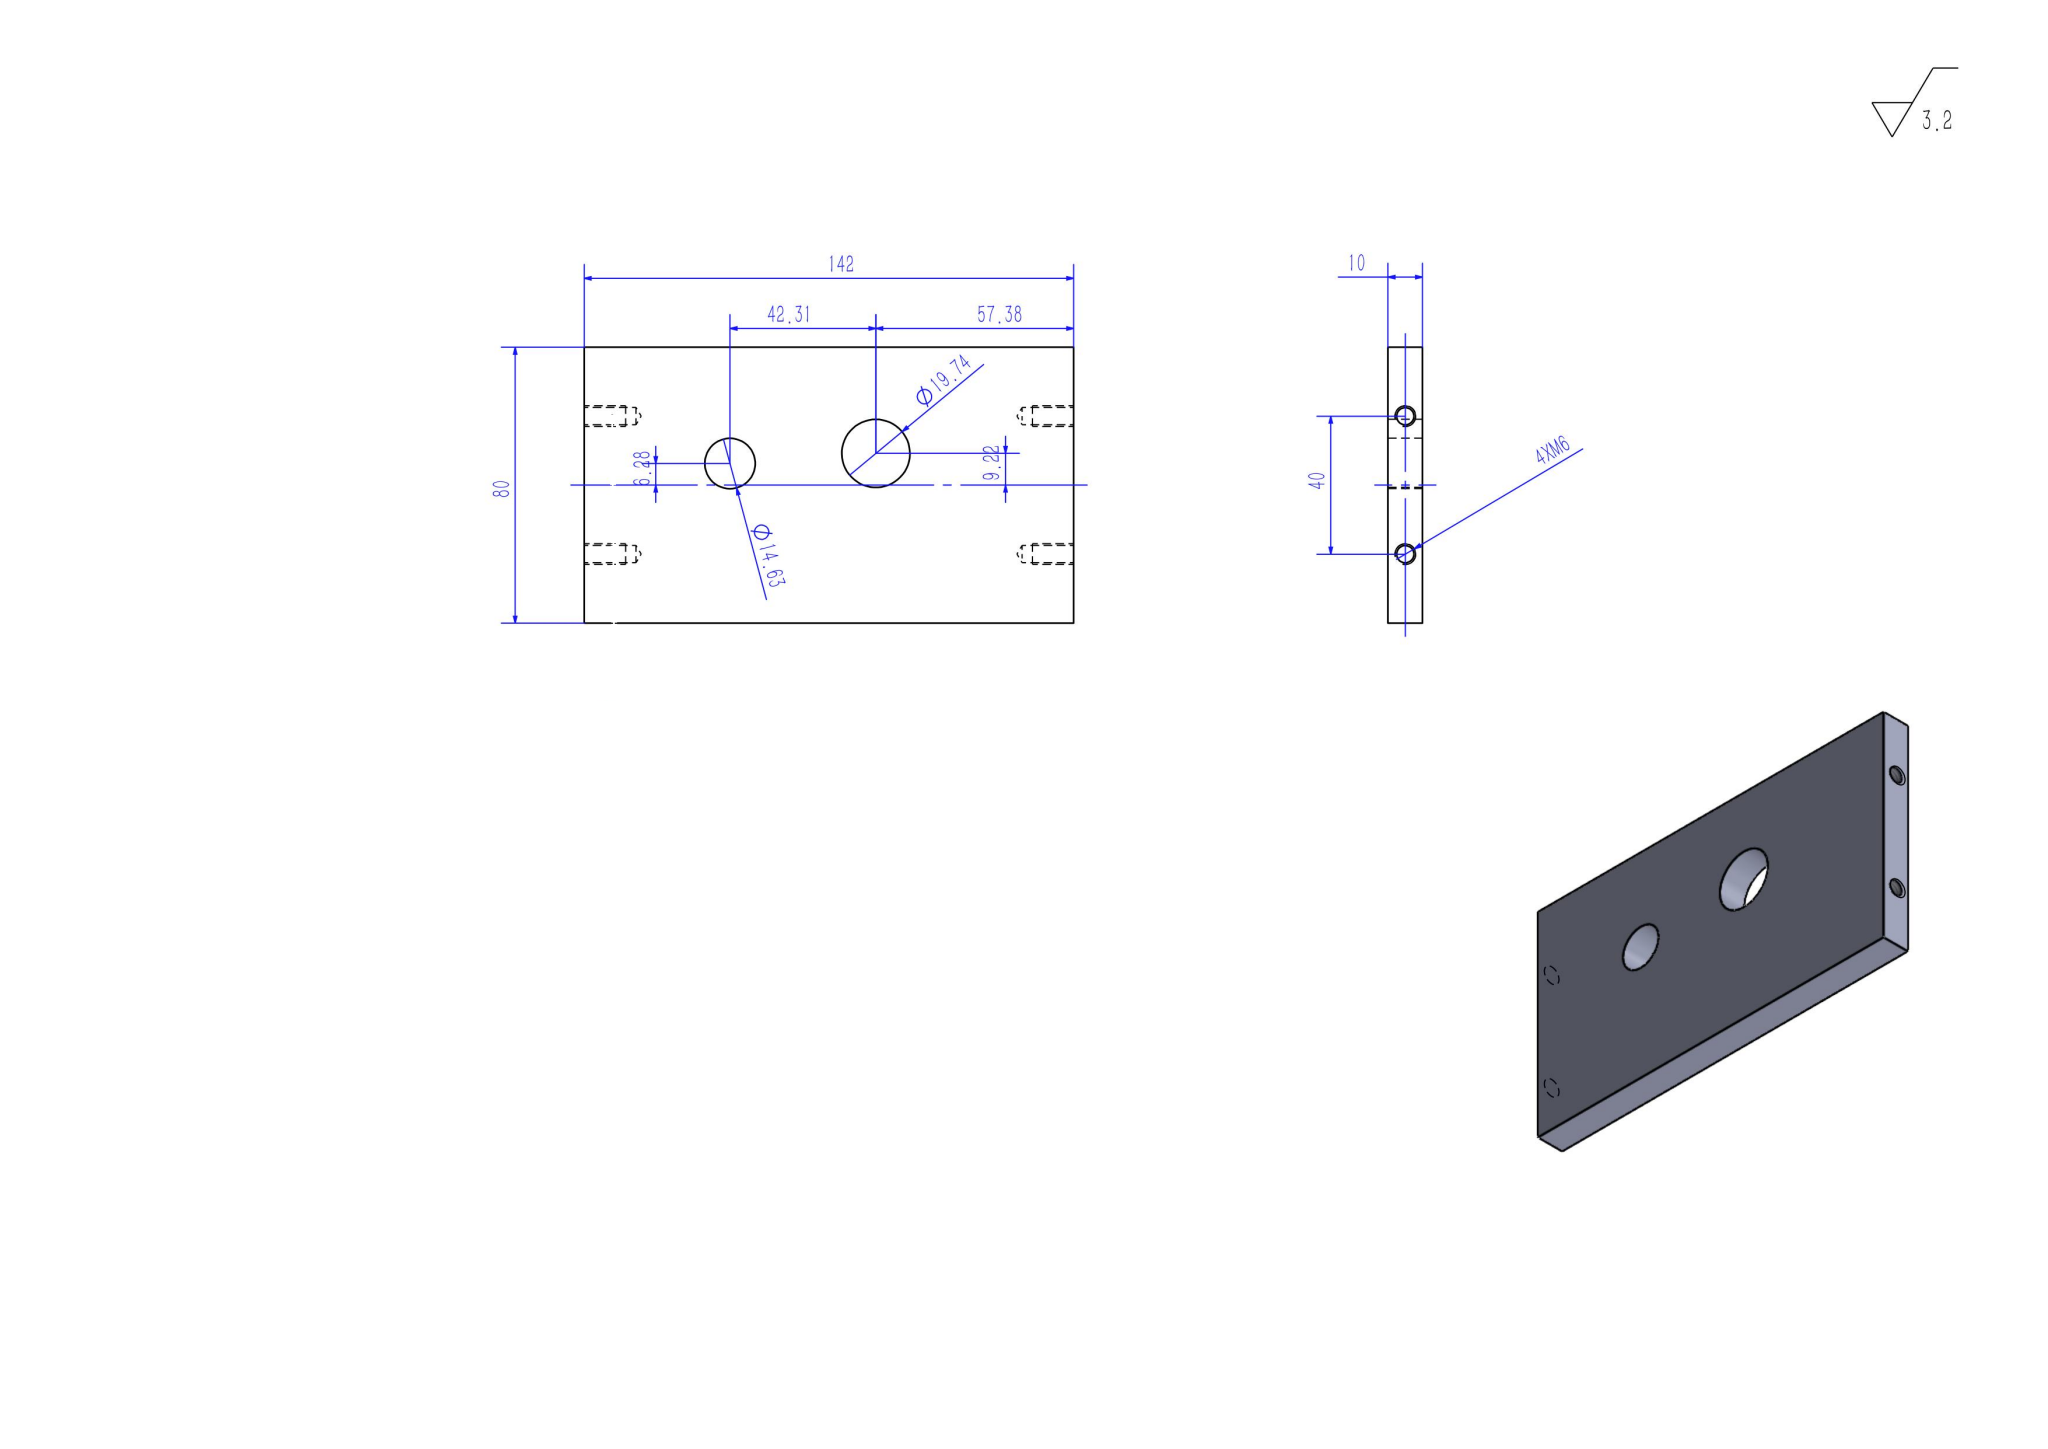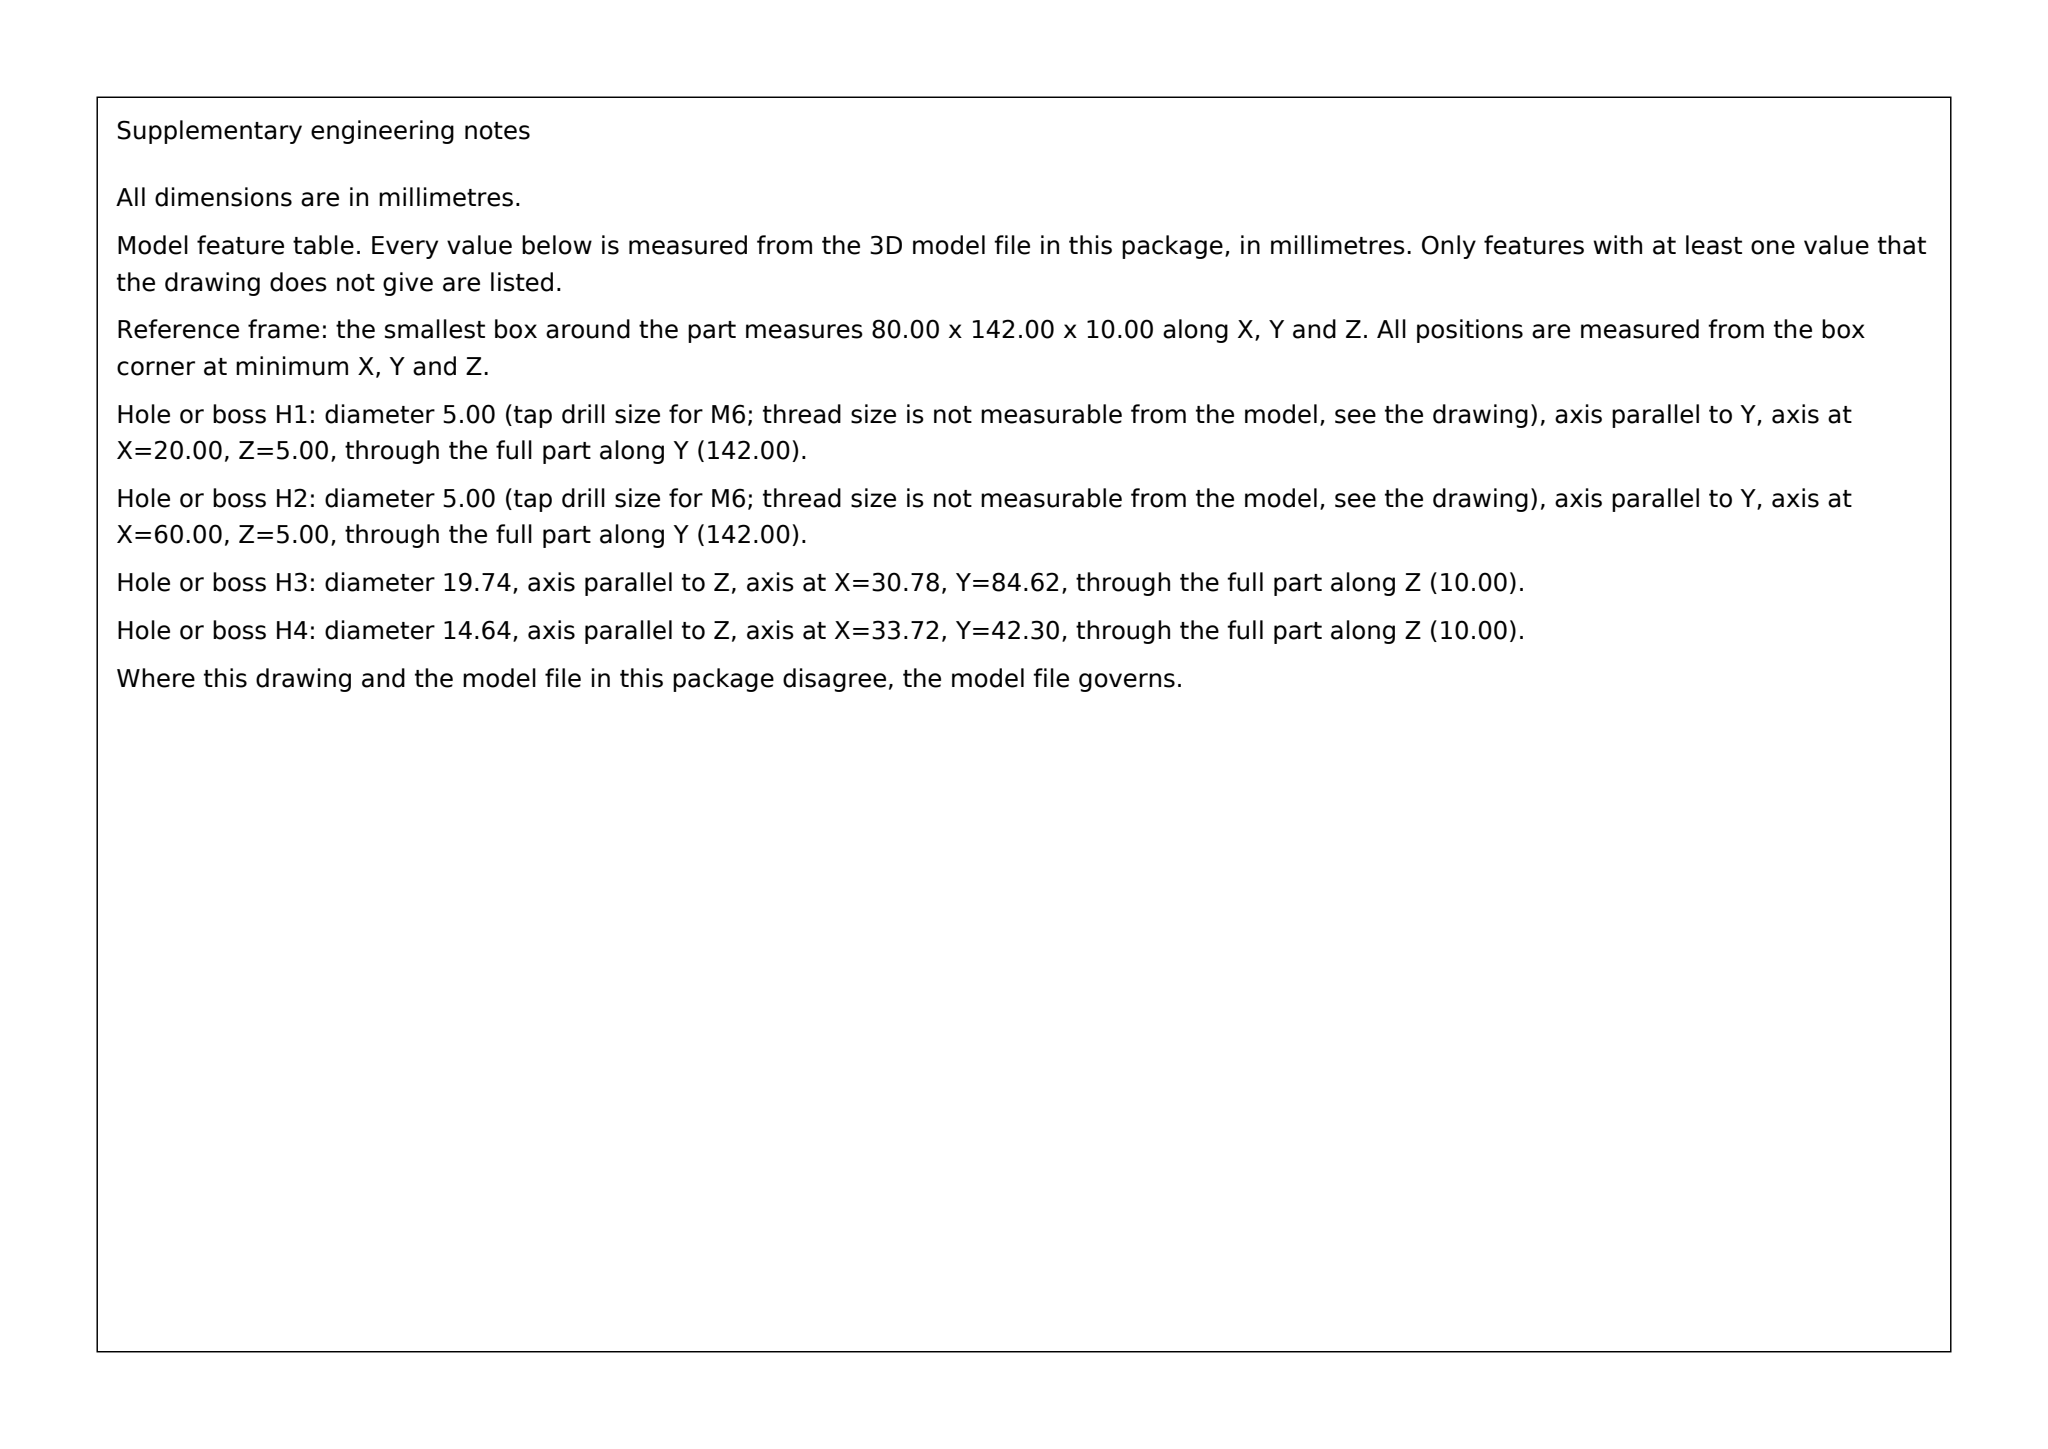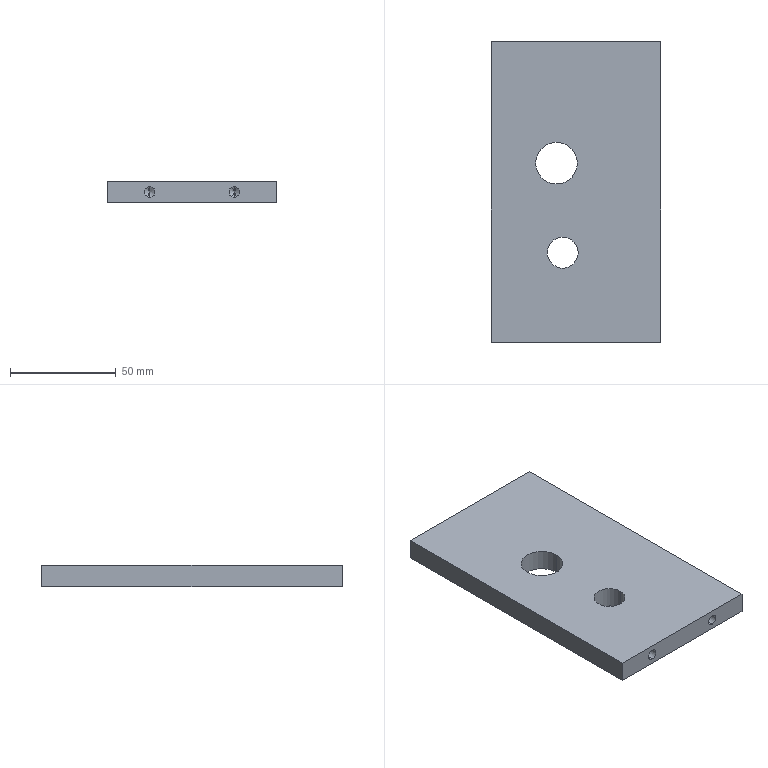Part | SolidWorks | mm | 1 solid | 26 faces | box 80 x 142 x 10 mm | volume 107639 mm3 | cylinder 12 | cone 8 | plane 6 | commonest cylinder face diameters 5 x8 14.633 x2 19.744 x2
build123d program:
from build123d import *

# Parameters (mm, degrees)
SKETCH1_W             = 80
SKETCH1_H             = 10
BOSS_EXTRUDE1_DEPTH   = 71
M6_TAPPED_HOLE1_D     = 5
M6_TAPPED_HOLE1_DEPTH = 15
M6_TAPPED_HOLE1_TIP   = 1.502
M6_TAPPED_HOLE2_D     = 5
M6_TAPPED_HOLE2_DEPTH = 15
M6_TAPPED_HOLE2_TIP   = 1.502
SKETCH6_R             = 7.317
SKETCH6_R_2           = 9.872
CUT_EXTRUDE1_DEPTH    = 80


with BuildPart() as part:
    # Sketch1 → Boss-Extrude1 (new, symmetric)
    with BuildSketch(Plane(origin=(0, 0, 0), x_dir=(1, 0, 0), z_dir=(0, 1, 0))):
        Rectangle(SKETCH1_W, SKETCH1_H)
    extrude(amount=BOSS_EXTRUDE1_DEPTH, both=True)

    # M6 Tapped Hole1
    with Locations(Plane(origin=(0, -71, 0), x_dir=(-1, 0, 0), z_dir=(0, -1, 0))):
        with Locations((20, 0), (-20, 0)):
            Hole(M6_TAPPED_HOLE1_D / 2, depth=M6_TAPPED_HOLE1_DEPTH)
            with Locations((0, 0, -(M6_TAPPED_HOLE1_DEPTH + M6_TAPPED_HOLE1_TIP / 2))):  # 118° drill point
                Cone(0, M6_TAPPED_HOLE1_D / 2, M6_TAPPED_HOLE1_TIP, mode=Mode.SUBTRACT)

    # M6 Tapped Hole2
    with Locations(Plane(origin=(0, 71, 0), x_dir=(1, 0, 0), z_dir=(0, 1, 0))):
        with Locations((-20, 0), (20, 0)):
            Hole(M6_TAPPED_HOLE2_D / 2, depth=M6_TAPPED_HOLE2_DEPTH)
            with Locations((0, 0, -(M6_TAPPED_HOLE2_DEPTH + M6_TAPPED_HOLE2_TIP / 2))):  # 118° drill point
                Cone(0, M6_TAPPED_HOLE2_D / 2, M6_TAPPED_HOLE2_TIP, mode=Mode.SUBTRACT)

    # Sketch6 → Cut-Extrude1 (cut)
    with BuildSketch(Plane(origin=(0, 0, -5), x_dir=(-1, 0, 0), z_dir=(0, 0, -1))):
        with Locations((6.284, -28.698)):
            Circle(SKETCH6_R)
        with Locations((9.217, 13.616)):
            Circle(SKETCH6_R_2)
    extrude(amount=-CUT_EXTRUDE1_DEPTH, mode=Mode.SUBTRACT)


solid = part.part
STEP:
#1=CARTESIAN_POINT('',(1.032,-28.698,5.));
#2=VERTEX_POINT('',#1);
#3=CARTESIAN_POINT('',(-13.601,-28.698,5.));
#4=VERTEX_POINT('',#3);
#5=CARTESIAN_POINT('',(-6.284,-28.698,5.));
#6=DIRECTION('',(0.,0.,-1.));
#7=DIRECTION('',(-1.,0.,0.));
#8=AXIS2_PLACEMENT_3D('',#5,#6,#7);
#9=CIRCLE('',#8,7.317);
#10=EDGE_CURVE('',#2,#4,#9,.T.);
#11=ORIENTED_EDGE('',*,*,#10,.F.);
#12=CARTESIAN_POINT('',(1.032,-28.698,-5.));
#13=VERTEX_POINT('',#12);
#14=CARTESIAN_POINT('',(1.032,-28.698,75.));
#15=DIRECTION('',(0.,0.,-1.));
#16=VECTOR('',#15,1000.);
#17=LINE('',#14,#16);
#18=EDGE_CURVE('',#2,#13,#17,.T.);
#19=ORIENTED_EDGE('',*,*,#18,.T.);
#20=CARTESIAN_POINT('',(-13.601,-28.698,-5.));
#21=VERTEX_POINT('',#20);
#22=CARTESIAN_POINT('',(-6.284,-28.698,-5.));
#23=DIRECTION('',(0.,0.,-1.));
#24=DIRECTION('',(-1.,0.,0.));
#25=AXIS2_PLACEMENT_3D('',#22,#23,#24);
#26=CIRCLE('',#25,7.317);
#27=EDGE_CURVE('',#13,#21,#26,.T.);
#28=ORIENTED_EDGE('',*,*,#27,.T.);
#29=CARTESIAN_POINT('',(-13.601,-28.698,75.));
#30=DIRECTION('',(0.,0.,-1.));
#31=VECTOR('',#30,1000.);
#32=LINE('',#29,#31);
#33=EDGE_CURVE('',#4,#21,#32,.T.);
#34=ORIENTED_EDGE('',*,*,#33,.F.);
#35=EDGE_LOOP('',(#11,#19,#28,#34));
#36=FACE_OUTER_BOUND('',#35,.T.);
#37=CARTESIAN_POINT('',(-6.284,-28.698,75.));
#38=DIRECTION('',(0.,0.,-1.));
#39=DIRECTION('',(-1.,0.,0.));
#40=AXIS2_PLACEMENT_3D('',#37,#38,#39);
#41=CYLINDRICAL_SURFACE('',#40,7.317);
#42=ADVANCED_FACE('',(#36),#41,.F.);
#43=CARTESIAN_POINT('',(0.6551,13.616,5.));
#44=VERTEX_POINT('',#43);
#45=CARTESIAN_POINT('',(-19.089,13.616,5.));
#46=VERTEX_POINT('',#45);
#47=CARTESIAN_POINT('',(-9.217,13.616,5.));
#48=DIRECTION('',(0.,0.,-1.));
#49=DIRECTION('',(-1.,0.,0.));
#50=AXIS2_PLACEMENT_3D('',#47,#48,#49);
#51=CIRCLE('',#50,9.872);
#52=EDGE_CURVE('',#44,#46,#51,.T.);
#53=ORIENTED_EDGE('',*,*,#52,.F.);
#54=CARTESIAN_POINT('',(0.6551,13.616,-5.));
#55=VERTEX_POINT('',#54);
#56=CARTESIAN_POINT('',(0.6551,13.616,75.));
#57=DIRECTION('',(0.,0.,-1.));
#58=VECTOR('',#57,1000.);
#59=LINE('',#56,#58);
#60=EDGE_CURVE('',#44,#55,#59,.T.);
#61=ORIENTED_EDGE('',*,*,#60,.T.);
#62=CARTESIAN_POINT('',(-19.089,13.616,-5.));
#63=VERTEX_POINT('',#62);
#64=CARTESIAN_POINT('',(-9.217,13.616,-5.));
#65=DIRECTION('',(0.,0.,-1.));
#66=DIRECTION('',(-1.,0.,0.));
#67=AXIS2_PLACEMENT_3D('',#64,#65,#66);
#68=CIRCLE('',#67,9.872);
#69=EDGE_CURVE('',#55,#63,#68,.T.);
#70=ORIENTED_EDGE('',*,*,#69,.T.);
#71=CARTESIAN_POINT('',(-19.089,13.616,75.));
#72=DIRECTION('',(0.,0.,-1.));
#73=VECTOR('',#72,1000.);
#74=LINE('',#71,#73);
#75=EDGE_CURVE('',#46,#63,#74,.T.);
#76=ORIENTED_EDGE('',*,*,#75,.F.);
#77=EDGE_LOOP('',(#53,#61,#70,#76));
#78=FACE_OUTER_BOUND('',#77,.T.);
#79=CARTESIAN_POINT('',(-9.217,13.616,75.));
#80=DIRECTION('',(0.,0.,-1.));
#81=DIRECTION('',(-1.,0.,0.));
#82=AXIS2_PLACEMENT_3D('',#79,#80,#81);
#83=CYLINDRICAL_SURFACE('',#82,9.872);
#84=ADVANCED_FACE('',(#78),#83,.F.);
#85=CARTESIAN_POINT('',(-20.,56.,-2.5));
#86=VERTEX_POINT('',#85);
#87=CARTESIAN_POINT('',(-20.,56.,2.5));
#88=VERTEX_POINT('',#87);
#89=CARTESIAN_POINT('',(-20.,56.,0.));
#90=DIRECTION('',(0.,1.,0.));
#91=DIRECTION('',(0.,0.,1.));
#92=AXIS2_PLACEMENT_3D('',#89,#90,#91);
#93=CIRCLE('',#92,2.5);
#94=EDGE_CURVE('',#86,#88,#93,.T.);
#95=ORIENTED_EDGE('',*,*,#94,.F.);
#96=CARTESIAN_POINT('',(-20.,71.,-2.5));
#97=VERTEX_POINT('',#96);
#98=CARTESIAN_POINT('',(-20.,71.,-2.5));
#99=DIRECTION('',(0.,1.,0.));
#100=VECTOR('',#99,1000.);
#101=LINE('',#98,#100);
#102=EDGE_CURVE('',#86,#97,#101,.T.);
#103=ORIENTED_EDGE('',*,*,#102,.T.);
#104=CARTESIAN_POINT('',(-20.,71.,2.5));
#105=VERTEX_POINT('',#104);
#106=CARTESIAN_POINT('',(-20.,71.,0.));
#107=DIRECTION('',(0.,1.,0.));
#108=DIRECTION('',(0.,0.,1.));
#109=AXIS2_PLACEMENT_3D('',#106,#107,#108);
#110=CIRCLE('',#109,2.5);
#111=EDGE_CURVE('',#97,#105,#110,.T.);
#112=ORIENTED_EDGE('',*,*,#111,.T.);
#113=CARTESIAN_POINT('',(-20.,71.,2.5));
#114=DIRECTION('',(0.,1.,0.));
#115=VECTOR('',#114,1000.);
#116=LINE('',#113,#115);
#117=EDGE_CURVE('',#88,#105,#116,.T.);
#118=ORIENTED_EDGE('',*,*,#117,.F.);
#119=EDGE_LOOP('',(#95,#103,#112,#118));
#120=FACE_OUTER_BOUND('',#119,.T.);
#121=CARTESIAN_POINT('',(-20.,71.,0.));
#122=DIRECTION('',(0.,1.,0.));
#123=DIRECTION('',(0.,0.,1.));
#124=AXIS2_PLACEMENT_3D('',#121,#122,#123);
#125=CYLINDRICAL_SURFACE('',#124,2.5);
#126=ADVANCED_FACE('',(#120),#125,.F.);
#127=CARTESIAN_POINT('',(-20.,54.498,0.));
#128=VERTEX_POINT('',#127);
#129=CARTESIAN_POINT('',(-20.,56.,2.5));
#130=DIRECTION('',(0.,0.515,0.8572));
#131=VECTOR('',#130,1000.);
#132=LINE('',#129,#131);
#133=EDGE_CURVE('',#128,#88,#132,.T.);
#134=ORIENTED_EDGE('',*,*,#133,.F.);
#135=CARTESIAN_POINT('',(-20.,56.,-2.5));
#136=DIRECTION('',(0.,0.515,-0.8572));
#137=VECTOR('',#136,1000.);
#138=LINE('',#135,#137);
#139=EDGE_CURVE('',#128,#86,#138,.T.);
#140=ORIENTED_EDGE('',*,*,#139,.T.);
#141=ORIENTED_EDGE('',*,*,#94,.T.);
#142=EDGE_LOOP('',(#134,#140,#141));
#143=FACE_OUTER_BOUND('',#142,.T.);
#144=CARTESIAN_POINT('',(-20.,56.,0.));
#145=DIRECTION('',(0.,1.,0.));
#146=DIRECTION('',(0.,0.,1.));
#147=AXIS2_PLACEMENT_3D('',#144,#145,#146);
#148=CONICAL_SURFACE('',#147,2.5,1.03);
#149=ADVANCED_FACE('',(#143),#148,.F.);
#150=CARTESIAN_POINT('',(20.,56.,-2.5));
#151=VERTEX_POINT('',#150);
#152=CARTESIAN_POINT('',(20.,56.,2.5));
#153=VERTEX_POINT('',#152);
#154=CARTESIAN_POINT('',(20.,56.,0.));
#155=DIRECTION('',(0.,1.,0.));
#156=DIRECTION('',(0.,0.,1.));
#157=AXIS2_PLACEMENT_3D('',#154,#155,#156);
#158=CIRCLE('',#157,2.5);
#159=EDGE_CURVE('',#151,#153,#158,.T.);
#160=ORIENTED_EDGE('',*,*,#159,.F.);
#161=CARTESIAN_POINT('',(20.,71.,-2.5));
#162=VERTEX_POINT('',#161);
#163=CARTESIAN_POINT('',(20.,71.,-2.5));
#164=DIRECTION('',(0.,1.,0.));
#165=VECTOR('',#164,1000.);
#166=LINE('',#163,#165);
#167=EDGE_CURVE('',#151,#162,#166,.T.);
#168=ORIENTED_EDGE('',*,*,#167,.T.);
#169=CARTESIAN_POINT('',(20.,71.,2.5));
#170=VERTEX_POINT('',#169);
#171=CARTESIAN_POINT('',(20.,71.,0.));
#172=DIRECTION('',(0.,1.,0.));
#173=DIRECTION('',(0.,0.,1.));
#174=AXIS2_PLACEMENT_3D('',#171,#172,#173);
#175=CIRCLE('',#174,2.5);
#176=EDGE_CURVE('',#162,#170,#175,.T.);
#177=ORIENTED_EDGE('',*,*,#176,.T.);
#178=CARTESIAN_POINT('',(20.,71.,2.5));
#179=DIRECTION('',(0.,1.,0.));
#180=VECTOR('',#179,1000.);
#181=LINE('',#178,#180);
#182=EDGE_CURVE('',#153,#170,#181,.T.);
#183=ORIENTED_EDGE('',*,*,#182,.F.);
#184=EDGE_LOOP('',(#160,#168,#177,#183));
#185=FACE_OUTER_BOUND('',#184,.T.);
#186=CARTESIAN_POINT('',(20.,71.,0.));
#187=DIRECTION('',(0.,1.,0.));
#188=DIRECTION('',(0.,0.,1.));
#189=AXIS2_PLACEMENT_3D('',#186,#187,#188);
#190=CYLINDRICAL_SURFACE('',#189,2.5);
#191=ADVANCED_FACE('',(#185),#190,.F.);
#192=CARTESIAN_POINT('',(20.,54.498,0.));
#193=VERTEX_POINT('',#192);
#194=CARTESIAN_POINT('',(20.,56.,2.5));
#195=DIRECTION('',(0.,0.515,0.8572));
#196=VECTOR('',#195,1000.);
#197=LINE('',#194,#196);
#198=EDGE_CURVE('',#193,#153,#197,.T.);
#199=ORIENTED_EDGE('',*,*,#198,.F.);
#200=CARTESIAN_POINT('',(20.,56.,-2.5));
#201=DIRECTION('',(0.,0.515,-0.8572));
#202=VECTOR('',#201,1000.);
#203=LINE('',#200,#202);
#204=EDGE_CURVE('',#193,#151,#203,.T.);
#205=ORIENTED_EDGE('',*,*,#204,.T.);
#206=ORIENTED_EDGE('',*,*,#159,.T.);
#207=EDGE_LOOP('',(#199,#205,#206));
#208=FACE_OUTER_BOUND('',#207,.T.);
#209=CARTESIAN_POINT('',(20.,56.,0.));
#210=DIRECTION('',(0.,1.,0.));
#211=DIRECTION('',(0.,0.,1.));
#212=AXIS2_PLACEMENT_3D('',#209,#210,#211);
#213=CONICAL_SURFACE('',#212,2.5,1.03);
#214=ADVANCED_FACE('',(#208),#213,.F.);
#215=CARTESIAN_POINT('',(-20.,-56.,2.5));
#216=VERTEX_POINT('',#215);
#217=CARTESIAN_POINT('',(-20.,-56.,-2.5));
#218=VERTEX_POINT('',#217);
#219=CARTESIAN_POINT('',(-20.,-56.,0.));
#220=DIRECTION('',(0.,-1.,0.));
#221=DIRECTION('',(0.,0.,-1.));
#222=AXIS2_PLACEMENT_3D('',#219,#220,#221);
#223=CIRCLE('',#222,2.5);
#224=EDGE_CURVE('',#216,#218,#223,.T.);
#225=ORIENTED_EDGE('',*,*,#224,.F.);
#226=CARTESIAN_POINT('',(-20.,-71.,2.5));
#227=VERTEX_POINT('',#226);
#228=CARTESIAN_POINT('',(-20.,-71.,2.5));
#229=DIRECTION('',(0.,-1.,0.));
#230=VECTOR('',#229,1000.);
#231=LINE('',#228,#230);
#232=EDGE_CURVE('',#216,#227,#231,.T.);
#233=ORIENTED_EDGE('',*,*,#232,.T.);
#234=CARTESIAN_POINT('',(-20.,-71.,-2.5));
#235=VERTEX_POINT('',#234);
#236=CARTESIAN_POINT('',(-20.,-71.,0.));
#237=DIRECTION('',(0.,-1.,0.));
#238=DIRECTION('',(0.,0.,-1.));
#239=AXIS2_PLACEMENT_3D('',#236,#237,#238);
#240=CIRCLE('',#239,2.5);
#241=EDGE_CURVE('',#227,#235,#240,.T.);
#242=ORIENTED_EDGE('',*,*,#241,.T.);
#243=CARTESIAN_POINT('',(-20.,-71.,-2.5));
#244=DIRECTION('',(0.,-1.,0.));
#245=VECTOR('',#244,1000.);
#246=LINE('',#243,#245);
#247=EDGE_CURVE('',#218,#235,#246,.T.);
#248=ORIENTED_EDGE('',*,*,#247,.F.);
#249=EDGE_LOOP('',(#225,#233,#242,#248));
#250=FACE_OUTER_BOUND('',#249,.T.);
#251=CARTESIAN_POINT('',(-20.,-71.,0.));
#252=DIRECTION('',(0.,-1.,0.));
#253=DIRECTION('',(0.,0.,-1.));
#254=AXIS2_PLACEMENT_3D('',#251,#252,#253);
#255=CYLINDRICAL_SURFACE('',#254,2.5);
#256=ADVANCED_FACE('',(#250),#255,.F.);
#257=CARTESIAN_POINT('',(-20.,-54.498,0.));
#258=VERTEX_POINT('',#257);
#259=CARTESIAN_POINT('',(-20.,-56.,-2.5));
#260=DIRECTION('',(0.,-0.515,-0.8572));
#261=VECTOR('',#260,1000.);
#262=LINE('',#259,#261);
#263=EDGE_CURVE('',#258,#218,#262,.T.);
#264=ORIENTED_EDGE('',*,*,#263,.F.);
#265=CARTESIAN_POINT('',(-20.,-56.,2.5));
#266=DIRECTION('',(0.,-0.515,0.8572));
#267=VECTOR('',#266,1000.);
#268=LINE('',#265,#267);
#269=EDGE_CURVE('',#258,#216,#268,.T.);
#270=ORIENTED_EDGE('',*,*,#269,.T.);
#271=ORIENTED_EDGE('',*,*,#224,.T.);
#272=EDGE_LOOP('',(#264,#270,#271));
#273=FACE_OUTER_BOUND('',#272,.T.);
#274=CARTESIAN_POINT('',(-20.,-56.,0.));
#275=DIRECTION('',(0.,-1.,0.));
#276=DIRECTION('',(0.,0.,-1.));
#277=AXIS2_PLACEMENT_3D('',#274,#275,#276);
#278=CONICAL_SURFACE('',#277,2.5,1.03);
#279=ADVANCED_FACE('',(#273),#278,.F.);
#280=CARTESIAN_POINT('',(20.,-56.,2.5));
#281=VERTEX_POINT('',#280);
#282=CARTESIAN_POINT('',(20.,-56.,-2.5));
#283=VERTEX_POINT('',#282);
#284=CARTESIAN_POINT('',(20.,-56.,0.));
#285=DIRECTION('',(0.,-1.,0.));
#286=DIRECTION('',(0.,0.,-1.));
#287=AXIS2_PLACEMENT_3D('',#284,#285,#286);
#288=CIRCLE('',#287,2.5);
#289=EDGE_CURVE('',#281,#283,#288,.T.);
#290=ORIENTED_EDGE('',*,*,#289,.F.);
#291=CARTESIAN_POINT('',(20.,-71.,2.5));
#292=VERTEX_POINT('',#291);
#293=CARTESIAN_POINT('',(20.,-71.,2.5));
#294=DIRECTION('',(0.,-1.,0.));
#295=VECTOR('',#294,1000.);
#296=LINE('',#293,#295);
#297=EDGE_CURVE('',#281,#292,#296,.T.);
#298=ORIENTED_EDGE('',*,*,#297,.T.);
#299=CARTESIAN_POINT('',(20.,-71.,-2.5));
#300=VERTEX_POINT('',#299);
#301=CARTESIAN_POINT('',(20.,-71.,0.));
#302=DIRECTION('',(0.,-1.,0.));
#303=DIRECTION('',(0.,0.,-1.));
#304=AXIS2_PLACEMENT_3D('',#301,#302,#303);
#305=CIRCLE('',#304,2.5);
#306=EDGE_CURVE('',#292,#300,#305,.T.);
#307=ORIENTED_EDGE('',*,*,#306,.T.);
#308=CARTESIAN_POINT('',(20.,-71.,-2.5));
#309=DIRECTION('',(0.,-1.,0.));
#310=VECTOR('',#309,1000.);
#311=LINE('',#308,#310);
#312=EDGE_CURVE('',#283,#300,#311,.T.);
#313=ORIENTED_EDGE('',*,*,#312,.F.);
#314=EDGE_LOOP('',(#290,#298,#307,#313));
#315=FACE_OUTER_BOUND('',#314,.T.);
#316=CARTESIAN_POINT('',(20.,-71.,0.));
#317=DIRECTION('',(0.,-1.,0.));
#318=DIRECTION('',(0.,0.,-1.));
#319=AXIS2_PLACEMENT_3D('',#316,#317,#318);
#320=CYLINDRICAL_SURFACE('',#319,2.5);
#321=ADVANCED_FACE('',(#315),#320,.F.);
#322=CARTESIAN_POINT('',(20.,-54.498,0.));
#323=VERTEX_POINT('',#322);
#324=CARTESIAN_POINT('',(20.,-56.,-2.5));
#325=DIRECTION('',(0.,-0.515,-0.8572));
#326=VECTOR('',#325,1000.);
#327=LINE('',#324,#326);
#328=EDGE_CURVE('',#323,#283,#327,.T.);
#329=ORIENTED_EDGE('',*,*,#328,.F.);
#330=CARTESIAN_POINT('',(20.,-56.,2.5));
#331=DIRECTION('',(0.,-0.515,0.8572));
#332=VECTOR('',#331,1000.);
#333=LINE('',#330,#332);
#334=EDGE_CURVE('',#323,#281,#333,.T.);
#335=ORIENTED_EDGE('',*,*,#334,.T.);
#336=ORIENTED_EDGE('',*,*,#289,.T.);
#337=EDGE_LOOP('',(#329,#335,#336));
#338=FACE_OUTER_BOUND('',#337,.T.);
#339=CARTESIAN_POINT('',(20.,-56.,0.));
#340=DIRECTION('',(0.,-1.,0.));
#341=DIRECTION('',(0.,0.,-1.));
#342=AXIS2_PLACEMENT_3D('',#339,#340,#341);
#343=CONICAL_SURFACE('',#342,2.5,1.03);
#344=ADVANCED_FACE('',(#338),#343,.F.);
#345=CARTESIAN_POINT('',(40.,-71.,5.));
#346=VERTEX_POINT('',#345);
#347=CARTESIAN_POINT('',(40.,-71.,-5.));
#348=VERTEX_POINT('',#347);
#349=CARTESIAN_POINT('',(40.,-71.,5.));
#350=DIRECTION('',(0.,0.,-1.));
#351=VECTOR('',#350,1000.);
#352=LINE('',#349,#351);
#353=EDGE_CURVE('',#346,#348,#352,.T.);
#354=ORIENTED_EDGE('',*,*,#353,.T.);
#355=CARTESIAN_POINT('',(40.,71.,-5.));
#356=VERTEX_POINT('',#355);
#357=CARTESIAN_POINT('',(40.,71.,-5.));
#358=DIRECTION('',(0.,-1.,0.));
#359=VECTOR('',#358,1000.);
#360=LINE('',#357,#359);
#361=EDGE_CURVE('',#356,#348,#360,.T.);
#362=ORIENTED_EDGE('',*,*,#361,.F.);
#363=CARTESIAN_POINT('',(40.,71.,5.));
#364=VERTEX_POINT('',#363);
#365=CARTESIAN_POINT('',(40.,71.,5.));
#366=DIRECTION('',(0.,0.,-1.));
#367=VECTOR('',#366,1000.);
#368=LINE('',#365,#367);
#369=EDGE_CURVE('',#364,#356,#368,.T.);
#370=ORIENTED_EDGE('',*,*,#369,.F.);
#371=CARTESIAN_POINT('',(40.,71.,5.));
#372=DIRECTION('',(0.,-1.,0.));
#373=VECTOR('',#372,1000.);
#374=LINE('',#371,#373);
#375=EDGE_CURVE('',#364,#346,#374,.T.);
#376=ORIENTED_EDGE('',*,*,#375,.T.);
#377=EDGE_LOOP('',(#354,#362,#370,#376));
#378=FACE_OUTER_BOUND('',#377,.T.);
#379=CARTESIAN_POINT('',(40.,71.,5.));
#380=DIRECTION('',(-1.,0.,0.));
#381=DIRECTION('',(0.,0.,1.));
#382=AXIS2_PLACEMENT_3D('',#379,#380,#381);
#383=PLANE('',#382);
#384=ADVANCED_FACE('',(#378),#383,.F.);
#385=CARTESIAN_POINT('',(-6.284,-28.698,-5.));
#386=DIRECTION('',(0.,0.,-1.));
#387=DIRECTION('',(-1.,0.,0.));
#388=AXIS2_PLACEMENT_3D('',#385,#386,#387);
#389=CIRCLE('',#388,7.317);
#390=EDGE_CURVE('',#21,#13,#389,.T.);
#391=ORIENTED_EDGE('',*,*,#390,.F.);
#392=ORIENTED_EDGE('',*,*,#27,.F.);
#393=EDGE_LOOP('',(#391,#392));
#394=FACE_BOUND('',#393,.T.);
#395=CARTESIAN_POINT('',(-9.217,13.616,-5.));
#396=DIRECTION('',(0.,0.,-1.));
#397=DIRECTION('',(-1.,0.,0.));
#398=AXIS2_PLACEMENT_3D('',#395,#396,#397);
#399=CIRCLE('',#398,9.872);
#400=EDGE_CURVE('',#63,#55,#399,.T.);
#401=ORIENTED_EDGE('',*,*,#400,.F.);
#402=ORIENTED_EDGE('',*,*,#69,.F.);
#403=EDGE_LOOP('',(#401,#402));
#404=FACE_BOUND('',#403,.T.);
#405=CARTESIAN_POINT('',(-40.,-71.,-5.));
#406=VERTEX_POINT('',#405);
#407=CARTESIAN_POINT('',(-40.,-71.,-5.));
#408=DIRECTION('',(-1.,0.,0.));
#409=VECTOR('',#408,1000.);
#410=LINE('',#407,#409);
#411=EDGE_CURVE('',#348,#406,#410,.T.);
#412=ORIENTED_EDGE('',*,*,#411,.T.);
#413=CARTESIAN_POINT('',(-40.,71.,-5.));
#414=VERTEX_POINT('',#413);
#415=CARTESIAN_POINT('',(-40.,71.,-5.));
#416=DIRECTION('',(0.,-1.,0.));
#417=VECTOR('',#416,1000.);
#418=LINE('',#415,#417);
#419=EDGE_CURVE('',#414,#406,#418,.T.);
#420=ORIENTED_EDGE('',*,*,#419,.F.);
#421=CARTESIAN_POINT('',(-40.,71.,-5.));
#422=DIRECTION('',(-1.,0.,0.));
#423=VECTOR('',#422,1000.);
#424=LINE('',#421,#423);
#425=EDGE_CURVE('',#356,#414,#424,.T.);
#426=ORIENTED_EDGE('',*,*,#425,.F.);
#427=ORIENTED_EDGE('',*,*,#361,.T.);
#428=EDGE_LOOP('',(#412,#420,#426,#427));
#429=FACE_OUTER_BOUND('',#428,.T.);
#430=CARTESIAN_POINT('',(-40.,71.,-5.));
#431=DIRECTION('',(0.,0.,1.));
#432=DIRECTION('',(1.,0.,0.));
#433=AXIS2_PLACEMENT_3D('',#430,#431,#432);
#434=PLANE('',#433);
#435=ADVANCED_FACE('',(#394,#404,#429),#434,.F.);
#436=CARTESIAN_POINT('',(-40.,-71.,5.));
#437=VERTEX_POINT('',#436);
#438=CARTESIAN_POINT('',(-40.,-71.,5.));
#439=DIRECTION('',(0.,0.,1.));
#440=VECTOR('',#439,1000.);
#441=LINE('',#438,#440);
#442=EDGE_CURVE('',#406,#437,#441,.T.);
#443=ORIENTED_EDGE('',*,*,#442,.T.);
#444=CARTESIAN_POINT('',(-40.,71.,5.));
#445=VERTEX_POINT('',#444);
#446=CARTESIAN_POINT('',(-40.,71.,5.));
#447=DIRECTION('',(0.,-1.,0.));
#448=VECTOR('',#447,1000.);
#449=LINE('',#446,#448);
#450=EDGE_CURVE('',#445,#437,#449,.T.);
#451=ORIENTED_EDGE('',*,*,#450,.F.);
#452=CARTESIAN_POINT('',(-40.,71.,5.));
#453=DIRECTION('',(0.,0.,1.));
#454=VECTOR('',#453,1000.);
#455=LINE('',#452,#454);
#456=EDGE_CURVE('',#414,#445,#455,.T.);
#457=ORIENTED_EDGE('',*,*,#456,.F.);
#458=ORIENTED_EDGE('',*,*,#419,.T.);
#459=EDGE_LOOP('',(#443,#451,#457,#458));
#460=FACE_OUTER_BOUND('',#459,.T.);
#461=CARTESIAN_POINT('',(-40.,71.,5.));
#462=DIRECTION('',(1.,0.,0.));
#463=DIRECTION('',(0.,0.,-1.));
#464=AXIS2_PLACEMENT_3D('',#461,#462,#463);
#465=PLANE('',#464);
#466=ADVANCED_FACE('',(#460),#465,.F.);
#467=CARTESIAN_POINT('',(-6.284,-28.698,5.));
#468=DIRECTION('',(0.,0.,-1.));
#469=DIRECTION('',(-1.,0.,0.));
#470=AXIS2_PLACEMENT_3D('',#467,#468,#469);
#471=CIRCLE('',#470,7.317);
#472=EDGE_CURVE('',#4,#2,#471,.T.);
#473=ORIENTED_EDGE('',*,*,#472,.T.);
#474=ORIENTED_EDGE('',*,*,#10,.T.);
#475=EDGE_LOOP('',(#473,#474));
#476=FACE_BOUND('',#475,.T.);
#477=CARTESIAN_POINT('',(-9.217,13.616,5.));
#478=DIRECTION('',(0.,0.,-1.));
#479=DIRECTION('',(-1.,0.,0.));
#480=AXIS2_PLACEMENT_3D('',#477,#478,#479);
#481=CIRCLE('',#480,9.872);
#482=EDGE_CURVE('',#46,#44,#481,.T.);
#483=ORIENTED_EDGE('',*,*,#482,.T.);
#484=ORIENTED_EDGE('',*,*,#52,.T.);
#485=EDGE_LOOP('',(#483,#484));
#486=FACE_BOUND('',#485,.T.);
#487=CARTESIAN_POINT('',(-40.,-71.,5.));
#488=DIRECTION('',(1.,0.,0.));
#489=VECTOR('',#488,1000.);
#490=LINE('',#487,#489);
#491=EDGE_CURVE('',#437,#346,#490,.T.);
#492=ORIENTED_EDGE('',*,*,#491,.T.);
#493=ORIENTED_EDGE('',*,*,#375,.F.);
#494=CARTESIAN_POINT('',(-40.,71.,5.));
#495=DIRECTION('',(1.,0.,0.));
#496=VECTOR('',#495,1000.);
#497=LINE('',#494,#496);
#498=EDGE_CURVE('',#445,#364,#497,.T.);
#499=ORIENTED_EDGE('',*,*,#498,.F.);
#500=ORIENTED_EDGE('',*,*,#450,.T.);
#501=EDGE_LOOP('',(#492,#493,#499,#500));
#502=FACE_OUTER_BOUND('',#501,.T.);
#503=CARTESIAN_POINT('',(-40.,71.,5.));
#504=DIRECTION('',(0.,0.,-1.));
#505=DIRECTION('',(-1.,0.,0.));
#506=AXIS2_PLACEMENT_3D('',#503,#504,#505);
#507=PLANE('',#506);
#508=ADVANCED_FACE('',(#476,#486,#502),#507,.F.);
#509=CARTESIAN_POINT('',(-20.,71.,0.));
#510=DIRECTION('',(0.,1.,0.));
#511=DIRECTION('',(0.,0.,1.));
#512=AXIS2_PLACEMENT_3D('',#509,#510,#511);
#513=CIRCLE('',#512,2.5);
#514=EDGE_CURVE('',#105,#97,#513,.T.);
#515=ORIENTED_EDGE('',*,*,#514,.F.);
#516=ORIENTED_EDGE('',*,*,#111,.F.);
#517=EDGE_LOOP('',(#515,#516));
#518=FACE_BOUND('',#517,.T.);
#519=CARTESIAN_POINT('',(20.,71.,0.));
#520=DIRECTION('',(0.,1.,0.));
#521=DIRECTION('',(0.,0.,1.));
#522=AXIS2_PLACEMENT_3D('',#519,#520,#521);
#523=CIRCLE('',#522,2.5);
#524=EDGE_CURVE('',#170,#162,#523,.T.);
#525=ORIENTED_EDGE('',*,*,#524,.F.);
#526=ORIENTED_EDGE('',*,*,#176,.F.);
#527=EDGE_LOOP('',(#525,#526));
#528=FACE_BOUND('',#527,.T.);
#529=ORIENTED_EDGE('',*,*,#369,.T.);
#530=ORIENTED_EDGE('',*,*,#425,.T.);
#531=ORIENTED_EDGE('',*,*,#456,.T.);
#532=ORIENTED_EDGE('',*,*,#498,.T.);
#533=EDGE_LOOP('',(#529,#530,#531,#532));
#534=FACE_OUTER_BOUND('',#533,.T.);
#535=CARTESIAN_POINT('',(0.,71.,0.));
#536=DIRECTION('',(0.,-1.,0.));
#537=DIRECTION('',(0.,0.,-1.));
#538=AXIS2_PLACEMENT_3D('',#535,#536,#537);
#539=PLANE('',#538);
#540=ADVANCED_FACE('',(#518,#528,#534),#539,.F.);
#541=CARTESIAN_POINT('',(-20.,-71.,0.));
#542=DIRECTION('',(0.,-1.,0.));
#543=DIRECTION('',(0.,0.,-1.));
#544=AXIS2_PLACEMENT_3D('',#541,#542,#543);
#545=CIRCLE('',#544,2.5);
#546=EDGE_CURVE('',#235,#227,#545,.T.);
#547=ORIENTED_EDGE('',*,*,#546,.F.);
#548=ORIENTED_EDGE('',*,*,#241,.F.);
#549=EDGE_LOOP('',(#547,#548));
#550=FACE_BOUND('',#549,.T.);
#551=CARTESIAN_POINT('',(20.,-71.,0.));
#552=DIRECTION('',(0.,-1.,0.));
#553=DIRECTION('',(0.,0.,-1.));
#554=AXIS2_PLACEMENT_3D('',#551,#552,#553);
#555=CIRCLE('',#554,2.5);
#556=EDGE_CURVE('',#300,#292,#555,.T.);
#557=ORIENTED_EDGE('',*,*,#556,.F.);
#558=ORIENTED_EDGE('',*,*,#306,.F.);
#559=EDGE_LOOP('',(#557,#558));
#560=FACE_BOUND('',#559,.T.);
#561=ORIENTED_EDGE('',*,*,#353,.F.);
#562=ORIENTED_EDGE('',*,*,#491,.F.);
#563=ORIENTED_EDGE('',*,*,#442,.F.);
#564=ORIENTED_EDGE('',*,*,#411,.F.);
#565=EDGE_LOOP('',(#561,#562,#563,#564));
#566=FACE_OUTER_BOUND('',#565,.T.);
#567=CARTESIAN_POINT('',(0.,-71.,0.));
#568=DIRECTION('',(0.,-1.,0.));
#569=DIRECTION('',(0.,0.,-1.));
#570=AXIS2_PLACEMENT_3D('',#567,#568,#569);
#571=PLANE('',#570);
#572=ADVANCED_FACE('',(#550,#560,#566),#571,.T.);
#573=ORIENTED_EDGE('',*,*,#334,.F.);
#574=ORIENTED_EDGE('',*,*,#328,.T.);
#575=CARTESIAN_POINT('',(20.,-56.,0.));
#576=DIRECTION('',(0.,-1.,0.));
#577=DIRECTION('',(0.,0.,-1.));
#578=AXIS2_PLACEMENT_3D('',#575,#576,#577);
#579=CIRCLE('',#578,2.5);
#580=EDGE_CURVE('',#283,#281,#579,.T.);
#581=ORIENTED_EDGE('',*,*,#580,.T.);
#582=EDGE_LOOP('',(#573,#574,#581));
#583=FACE_OUTER_BOUND('',#582,.T.);
#584=CARTESIAN_POINT('',(20.,-56.,0.));
#585=DIRECTION('',(0.,-1.,0.));
#586=DIRECTION('',(0.,0.,-1.));
#587=AXIS2_PLACEMENT_3D('',#584,#585,#586);
#588=CONICAL_SURFACE('',#587,2.5,1.03);
#589=ADVANCED_FACE('',(#583),#588,.F.);
#590=ORIENTED_EDGE('',*,*,#297,.F.);
#591=ORIENTED_EDGE('',*,*,#580,.F.);
#592=ORIENTED_EDGE('',*,*,#312,.T.);
#593=ORIENTED_EDGE('',*,*,#556,.T.);
#594=EDGE_LOOP('',(#590,#591,#592,#593));
#595=FACE_OUTER_BOUND('',#594,.T.);
#596=CARTESIAN_POINT('',(20.,-71.,0.));
#597=DIRECTION('',(0.,-1.,0.));
#598=DIRECTION('',(0.,0.,-1.));
#599=AXIS2_PLACEMENT_3D('',#596,#597,#598);
#600=CYLINDRICAL_SURFACE('',#599,2.5);
#601=ADVANCED_FACE('',(#595),#600,.F.);
#602=ORIENTED_EDGE('',*,*,#269,.F.);
#603=ORIENTED_EDGE('',*,*,#263,.T.);
#604=CARTESIAN_POINT('',(-20.,-56.,0.));
#605=DIRECTION('',(0.,-1.,0.));
#606=DIRECTION('',(0.,0.,-1.));
#607=AXIS2_PLACEMENT_3D('',#604,#605,#606);
#608=CIRCLE('',#607,2.5);
#609=EDGE_CURVE('',#218,#216,#608,.T.);
#610=ORIENTED_EDGE('',*,*,#609,.T.);
#611=EDGE_LOOP('',(#602,#603,#610));
#612=FACE_OUTER_BOUND('',#611,.T.);
#613=CARTESIAN_POINT('',(-20.,-56.,0.));
#614=DIRECTION('',(0.,-1.,0.));
#615=DIRECTION('',(0.,0.,-1.));
#616=AXIS2_PLACEMENT_3D('',#613,#614,#615);
#617=CONICAL_SURFACE('',#616,2.5,1.03);
#618=ADVANCED_FACE('',(#612),#617,.F.);
#619=ORIENTED_EDGE('',*,*,#232,.F.);
#620=ORIENTED_EDGE('',*,*,#609,.F.);
#621=ORIENTED_EDGE('',*,*,#247,.T.);
#622=ORIENTED_EDGE('',*,*,#546,.T.);
#623=EDGE_LOOP('',(#619,#620,#621,#622));
#624=FACE_OUTER_BOUND('',#623,.T.);
#625=CARTESIAN_POINT('',(-20.,-71.,0.));
#626=DIRECTION('',(0.,-1.,0.));
#627=DIRECTION('',(0.,0.,-1.));
#628=AXIS2_PLACEMENT_3D('',#625,#626,#627);
#629=CYLINDRICAL_SURFACE('',#628,2.5);
#630=ADVANCED_FACE('',(#624),#629,.F.);
#631=ORIENTED_EDGE('',*,*,#204,.F.);
#632=ORIENTED_EDGE('',*,*,#198,.T.);
#633=CARTESIAN_POINT('',(20.,56.,0.));
#634=DIRECTION('',(0.,1.,0.));
#635=DIRECTION('',(0.,0.,1.));
#636=AXIS2_PLACEMENT_3D('',#633,#634,#635);
#637=CIRCLE('',#636,2.5);
#638=EDGE_CURVE('',#153,#151,#637,.T.);
#639=ORIENTED_EDGE('',*,*,#638,.T.);
#640=EDGE_LOOP('',(#631,#632,#639));
#641=FACE_OUTER_BOUND('',#640,.T.);
#642=CARTESIAN_POINT('',(20.,56.,0.));
#643=DIRECTION('',(0.,1.,0.));
#644=DIRECTION('',(0.,0.,1.));
#645=AXIS2_PLACEMENT_3D('',#642,#643,#644);
#646=CONICAL_SURFACE('',#645,2.5,1.03);
#647=ADVANCED_FACE('',(#641),#646,.F.);
#648=ORIENTED_EDGE('',*,*,#167,.F.);
#649=ORIENTED_EDGE('',*,*,#638,.F.);
#650=ORIENTED_EDGE('',*,*,#182,.T.);
#651=ORIENTED_EDGE('',*,*,#524,.T.);
#652=EDGE_LOOP('',(#648,#649,#650,#651));
#653=FACE_OUTER_BOUND('',#652,.T.);
#654=CARTESIAN_POINT('',(20.,71.,0.));
#655=DIRECTION('',(0.,1.,0.));
#656=DIRECTION('',(0.,0.,1.));
#657=AXIS2_PLACEMENT_3D('',#654,#655,#656);
#658=CYLINDRICAL_SURFACE('',#657,2.5);
#659=ADVANCED_FACE('',(#653),#658,.F.);
#660=ORIENTED_EDGE('',*,*,#139,.F.);
#661=ORIENTED_EDGE('',*,*,#133,.T.);
#662=CARTESIAN_POINT('',(-20.,56.,0.));
#663=DIRECTION('',(0.,1.,0.));
#664=DIRECTION('',(0.,0.,1.));
#665=AXIS2_PLACEMENT_3D('',#662,#663,#664);
#666=CIRCLE('',#665,2.5);
#667=EDGE_CURVE('',#88,#86,#666,.T.);
#668=ORIENTED_EDGE('',*,*,#667,.T.);
#669=EDGE_LOOP('',(#660,#661,#668));
#670=FACE_OUTER_BOUND('',#669,.T.);
#671=CARTESIAN_POINT('',(-20.,56.,0.));
#672=DIRECTION('',(0.,1.,0.));
#673=DIRECTION('',(0.,0.,1.));
#674=AXIS2_PLACEMENT_3D('',#671,#672,#673);
#675=CONICAL_SURFACE('',#674,2.5,1.03);
#676=ADVANCED_FACE('',(#670),#675,.F.);
#677=ORIENTED_EDGE('',*,*,#102,.F.);
#678=ORIENTED_EDGE('',*,*,#667,.F.);
#679=ORIENTED_EDGE('',*,*,#117,.T.);
#680=ORIENTED_EDGE('',*,*,#514,.T.);
#681=EDGE_LOOP('',(#677,#678,#679,#680));
#682=FACE_OUTER_BOUND('',#681,.T.);
#683=CARTESIAN_POINT('',(-20.,71.,0.));
#684=DIRECTION('',(0.,1.,0.));
#685=DIRECTION('',(0.,0.,1.));
#686=AXIS2_PLACEMENT_3D('',#683,#684,#685);
#687=CYLINDRICAL_SURFACE('',#686,2.5);
#688=ADVANCED_FACE('',(#682),#687,.F.);
#689=ORIENTED_EDGE('',*,*,#60,.F.);
#690=ORIENTED_EDGE('',*,*,#482,.F.);
#691=ORIENTED_EDGE('',*,*,#75,.T.);
#692=ORIENTED_EDGE('',*,*,#400,.T.);
#693=EDGE_LOOP('',(#689,#690,#691,#692));
#694=FACE_OUTER_BOUND('',#693,.T.);
#695=CARTESIAN_POINT('',(-9.217,13.616,75.));
#696=DIRECTION('',(0.,0.,-1.));
#697=DIRECTION('',(-1.,0.,0.));
#698=AXIS2_PLACEMENT_3D('',#695,#696,#697);
#699=CYLINDRICAL_SURFACE('',#698,9.872);
#700=ADVANCED_FACE('',(#694),#699,.F.);
#701=ORIENTED_EDGE('',*,*,#18,.F.);
#702=ORIENTED_EDGE('',*,*,#472,.F.);
#703=ORIENTED_EDGE('',*,*,#33,.T.);
#704=ORIENTED_EDGE('',*,*,#390,.T.);
#705=EDGE_LOOP('',(#701,#702,#703,#704));
#706=FACE_OUTER_BOUND('',#705,.T.);
#707=CARTESIAN_POINT('',(-6.284,-28.698,75.));
#708=DIRECTION('',(0.,0.,-1.));
#709=DIRECTION('',(-1.,0.,0.));
#710=AXIS2_PLACEMENT_3D('',#707,#708,#709);
#711=CYLINDRICAL_SURFACE('',#710,7.317);
#712=ADVANCED_FACE('',(#706),#711,.F.);
#713=CLOSED_SHELL('',(#42,#84,#126,#149,#191,#214,#256,#279,#321,#344,#384,#435,#466,#508,#540,#572,#589,#601,#618,#630,#647,#659,#676,#688,#700,#712));
#714=MANIFOLD_SOLID_BREP('',#713);
#715=CARTESIAN_POINT('',(0.,0.,0.));
#716=DIRECTION('',(0.,0.,1.));
#717=DIRECTION('',(1.,0.,0.));
#718=AXIS2_PLACEMENT_3D('',#715,#716,#717);
#719=(LENGTH_UNIT()NAMED_UNIT(*)SI_UNIT(.MILLI.,.METRE.));
#720=UNCERTAINTY_MEASURE_WITH_UNIT(LENGTH_MEASURE(0.00001),#719,'','');
#721=(NAMED_UNIT(*)PLANE_ANGLE_UNIT()SI_UNIT($,.RADIAN.));
#722=(NAMED_UNIT(*)SI_UNIT($,.STERADIAN.)SOLID_ANGLE_UNIT());
#723=(GEOMETRIC_REPRESENTATION_CONTEXT(3)GLOBAL_UNCERTAINTY_ASSIGNED_CONTEXT((#720))GLOBAL_UNIT_ASSIGNED_CONTEXT((#719,#721,#722))REPRESENTATION_CONTEXT('',''));
#724=ADVANCED_BREP_SHAPE_REPRESENTATION('',(#714,#718),#723);